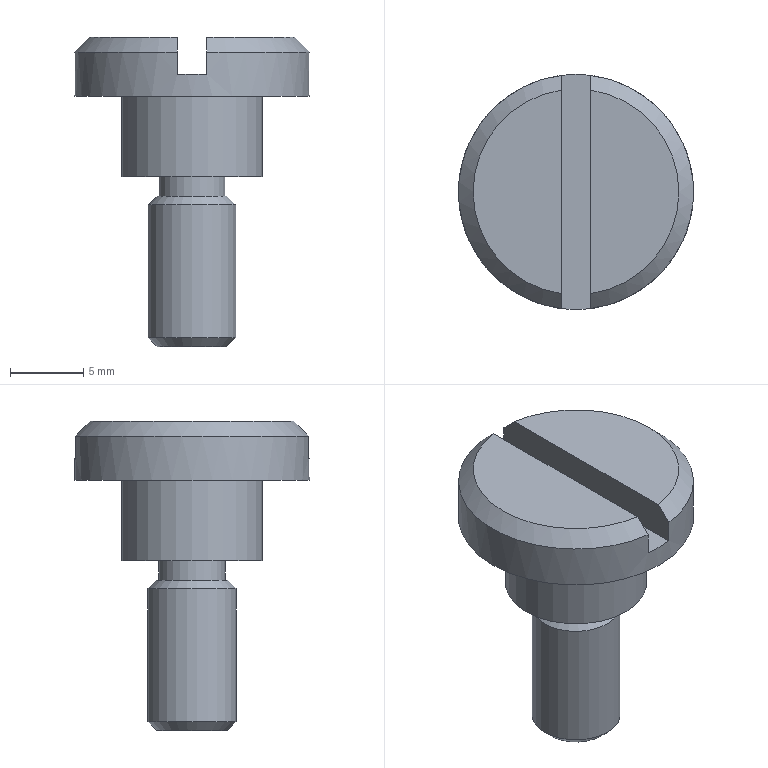Component | NX | DRILL_BUSH_SCREW | 1 solid | 17 faces | volume 1405 mm3 | plane 9 | cylinder 4 | cone 4 | commonest cylinder face diameters 6 x1 4.5 x1 9.6 x1 16 x1